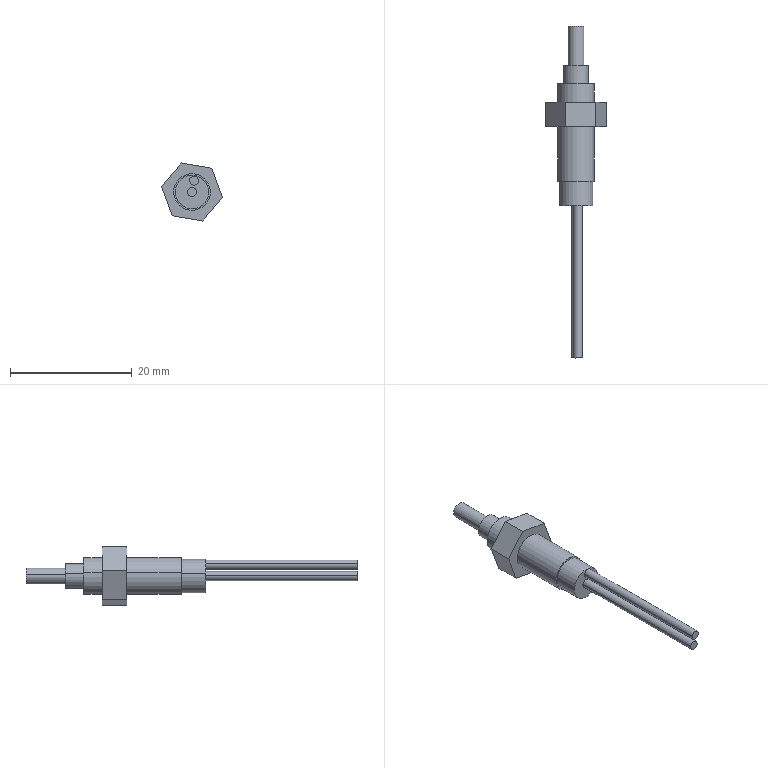Component | SolidWorks | 610FiberOptic-1 | 1 solid | 29 faces | box 10.01 x 54.5 x 9.54 mm | volume 863 mm3 | plane 15 | cylinder 14 | commonest cylinder face diameters 1.5 x4 6 x4 5.5 x2 4 x2 2.6 x2
build123d program:
from build123d import *

# Parameters (mm, degrees)
SKETCH1_R           = 3
BOSS_EXTRUDE1_DEPTH = 20
SKETCH2_R           = 2
BOSS_EXTRUDE2_DEPTH = 3
SKETCH3_R           = 0.75
BOSS_EXTRUDE3_DEPTH = 25
BOSS_EXTRUDE4_DEPTH = 4
SKETCH5_R           = 1.3
BOSS_EXTRUDE5_DEPTH = 11
CUT_EXTRUDE1_START  = -4
SKETCH6_R           = 3
SKETCH6_R_2         = 2.75
CUT_EXTRUDE1_DEPTH  = 4
CUT_EXTRUDE2_START  = -4.5
SKETCH7_R           = 1.3
CUT_EXTRUDE2_DEPTH  = 4.5


with BuildPart() as part:
    # Sketch1 → Boss-Extrude1 (new body)
    with BuildSketch(Plane.XY):
        Circle(SKETCH1_R)
    extrude(amount=BOSS_EXTRUDE1_DEPTH)

    # Sketch2 → Boss-Extrude2 (add)
    with BuildSketch(Plane(origin=(0, 0, 0), x_dir=(-1, 0, 0), z_dir=(0, 0, -1))):
        with Locations(Location((0, 0, 0), (0, 0, 180))):
            Circle(SKETCH2_R)
    extrude(amount=BOSS_EXTRUDE2_DEPTH)

    # Sketch3 → Boss-Extrude3 (add)
    with BuildSketch(Plane.XY.offset(20)):
        with Locations((0, 1.9)):
            Circle(SKETCH3_R)
        Circle(SKETCH3_R)
    extrude(amount=BOSS_EXTRUDE3_DEPTH)

    # Sketch4 → Boss-Extrude4 (add)
    with BuildSketch(Plane(origin=(0, 0, 3), x_dir=(-1, 0, 0), z_dir=(0, 0, -1))):
        Polygon((2.54, 4.4), (-2.54, 4.4), (-5.081, 0), (-2.54, -4.4), (2.54, -4.4), (5.081, 0), align=None)
    extrude(amount=-BOSS_EXTRUDE4_DEPTH)

    # Sketch5 → Boss-Extrude5 (add)
    with BuildSketch(Plane(origin=(0, 0, -3), x_dir=(-1, 0, 0), z_dir=(0, 0, -1))):
        Circle(SKETCH5_R)
    extrude(amount=BOSS_EXTRUDE5_DEPTH)

    # Sketch6 → Cut-Extrude1 (cut)
    with BuildSketch(Plane.XY.offset(20).offset(CUT_EXTRUDE1_START)):
        with Locations(Location((0, 0, 0), (0, 0, 180))):
            Circle(SKETCH6_R)
        Circle(SKETCH6_R_2, mode=Mode.SUBTRACT)
    extrude(amount=CUT_EXTRUDE1_DEPTH, mode=Mode.SUBTRACT)

    # Sketch7 → Cut-Extrude2 (cut)
    with BuildSketch(Plane(origin=(0, 0, -14), x_dir=(-1, 0, 0), z_dir=(0, 0, -1)).offset(CUT_EXTRUDE2_START)):
        Circle(SKETCH7_R)
    extrude(amount=CUT_EXTRUDE2_DEPTH, mode=Mode.SUBTRACT)


solid = part.part

# Placed as in the assembly
solid = solid.moved(Location((-18.365, -4.305, 118.579), (90, 0, -9.806)))
STEP:
#1=CARTESIAN_POINT('',(-0.6939,-1.941,4.663));
#2=VERTEX_POINT('',#1);
#3=CARTESIAN_POINT('',(-0.7521,-1.941,4.673));
#4=VERTEX_POINT('',#3);
#5=CARTESIAN_POINT('',(-0.723,-1.941,4.668));
#6=DIRECTION('',(-0.,-1.,-0.));
#7=DIRECTION('',(0.9854,0.,-0.1703));
#8=AXIS2_PLACEMENT_3D('',#5,#6,#7);
#9=CIRCLE('',#8,0.02953);
#10=EDGE_CURVE('',#2,#4,#9,.T.);
#11=ORIENTED_EDGE('',*,*,#10,.F.);
#12=CARTESIAN_POINT('',(-0.6939,-0.9569,4.663));
#13=VERTEX_POINT('',#12);
#14=CARTESIAN_POINT('',(-0.6939,-1.941,4.663));
#15=DIRECTION('',(0.,1.,0.));
#16=VECTOR('',#15,39.37);
#17=LINE('',#14,#16);
#18=EDGE_CURVE('',#2,#13,#17,.T.);
#19=ORIENTED_EDGE('',*,*,#18,.T.);
#20=CARTESIAN_POINT('',(-0.7521,-0.9569,4.673));
#21=VERTEX_POINT('',#20);
#22=CARTESIAN_POINT('',(-0.723,-0.9569,4.668));
#23=DIRECTION('',(-0.,-1.,-0.));
#24=DIRECTION('',(0.9854,0.,-0.1703));
#25=AXIS2_PLACEMENT_3D('',#22,#23,#24);
#26=CIRCLE('',#25,0.02953);
#27=EDGE_CURVE('',#13,#21,#26,.T.);
#28=ORIENTED_EDGE('',*,*,#27,.T.);
#29=CARTESIAN_POINT('',(-0.7521,-1.941,4.673));
#30=DIRECTION('',(0.,1.,0.));
#31=VECTOR('',#30,39.37);
#32=LINE('',#29,#31);
#33=EDGE_CURVE('',#4,#21,#32,.T.);
#34=ORIENTED_EDGE('',*,*,#33,.F.);
#35=EDGE_LOOP('',(#11,#19,#28,#34));
#36=FACE_OUTER_BOUND('',#35,.T.);
#37=CARTESIAN_POINT('',(-0.723,-1.941,4.668));
#38=DIRECTION('',(0.,1.,0.));
#39=DIRECTION('',(-0.9854,0.,0.1703));
#40=AXIS2_PLACEMENT_3D('',#37,#38,#39);
#41=CYLINDRICAL_SURFACE('',#40,0.02953);
#42=ADVANCED_FACE('',(#36),#41,.T.);
#43=CARTESIAN_POINT('',(-0.6812,-1.941,4.737));
#44=VERTEX_POINT('',#43);
#45=CARTESIAN_POINT('',(-0.7394,-1.941,4.747));
#46=VERTEX_POINT('',#45);
#47=CARTESIAN_POINT('',(-0.7103,-1.941,4.742));
#48=DIRECTION('',(-0.,-1.,-0.));
#49=DIRECTION('',(0.9854,0.,-0.1703));
#50=AXIS2_PLACEMENT_3D('',#47,#48,#49);
#51=CIRCLE('',#50,0.02953);
#52=EDGE_CURVE('',#44,#46,#51,.T.);
#53=ORIENTED_EDGE('',*,*,#52,.F.);
#54=CARTESIAN_POINT('',(-0.6812,-0.9569,4.737));
#55=VERTEX_POINT('',#54);
#56=CARTESIAN_POINT('',(-0.6812,-1.941,4.737));
#57=DIRECTION('',(0.,1.,0.));
#58=VECTOR('',#57,39.37);
#59=LINE('',#56,#58);
#60=EDGE_CURVE('',#44,#55,#59,.T.);
#61=ORIENTED_EDGE('',*,*,#60,.T.);
#62=CARTESIAN_POINT('',(-0.7394,-0.9569,4.747));
#63=VERTEX_POINT('',#62);
#64=CARTESIAN_POINT('',(-0.7103,-0.9569,4.742));
#65=DIRECTION('',(-0.,-1.,-0.));
#66=DIRECTION('',(0.9854,0.,-0.1703));
#67=AXIS2_PLACEMENT_3D('',#64,#65,#66);
#68=CIRCLE('',#67,0.02953);
#69=EDGE_CURVE('',#55,#63,#68,.T.);
#70=ORIENTED_EDGE('',*,*,#69,.T.);
#71=CARTESIAN_POINT('',(-0.7394,-1.941,4.747));
#72=DIRECTION('',(0.,1.,0.));
#73=VECTOR('',#72,39.37);
#74=LINE('',#71,#73);
#75=EDGE_CURVE('',#46,#63,#74,.T.);
#76=ORIENTED_EDGE('',*,*,#75,.F.);
#77=EDGE_LOOP('',(#53,#61,#70,#76));
#78=FACE_OUTER_BOUND('',#77,.T.);
#79=CARTESIAN_POINT('',(-0.7103,-1.941,4.742));
#80=DIRECTION('',(0.,1.,0.));
#81=DIRECTION('',(-0.9854,0.,0.1703));
#82=AXIS2_PLACEMENT_3D('',#79,#80,#81);
#83=CYLINDRICAL_SURFACE('',#82,0.02953);
#84=ADVANCED_FACE('',(#78),#83,.T.);
#85=CARTESIAN_POINT('',(-0.6163,-0.7994,4.65));
#86=VERTEX_POINT('',#85);
#87=CARTESIAN_POINT('',(-0.8297,-0.7994,4.687));
#88=VERTEX_POINT('',#87);
#89=CARTESIAN_POINT('',(-0.723,-0.7994,4.668));
#90=DIRECTION('',(-0.,-1.,-0.));
#91=DIRECTION('',(0.9854,0.,-0.1703));
#92=AXIS2_PLACEMENT_3D('',#89,#90,#91);
#93=CIRCLE('',#92,0.1083);
#94=EDGE_CURVE('',#86,#88,#93,.T.);
#95=ORIENTED_EDGE('',*,*,#94,.T.);
#96=CARTESIAN_POINT('',(-0.8297,-0.9569,4.687));
#97=VERTEX_POINT('',#96);
#98=CARTESIAN_POINT('',(-0.8297,-0.7994,4.687));
#99=DIRECTION('',(-0.,-1.,-0.));
#100=VECTOR('',#99,39.37);
#101=LINE('',#98,#100);
#102=EDGE_CURVE('',#88,#97,#101,.T.);
#103=ORIENTED_EDGE('',*,*,#102,.T.);
#104=CARTESIAN_POINT('',(-0.6163,-0.9569,4.65));
#105=VERTEX_POINT('',#104);
#106=CARTESIAN_POINT('',(-0.723,-0.9569,4.668));
#107=DIRECTION('',(-0.,-1.,-0.));
#108=DIRECTION('',(0.9854,0.,-0.1703));
#109=AXIS2_PLACEMENT_3D('',#106,#107,#108);
#110=CIRCLE('',#109,0.1083);
#111=EDGE_CURVE('',#105,#97,#110,.T.);
#112=ORIENTED_EDGE('',*,*,#111,.F.);
#113=CARTESIAN_POINT('',(-0.6163,-0.7994,4.65));
#114=DIRECTION('',(-0.,-1.,-0.));
#115=VECTOR('',#114,39.37);
#116=LINE('',#113,#115);
#117=EDGE_CURVE('',#86,#105,#116,.T.);
#118=ORIENTED_EDGE('',*,*,#117,.F.);
#119=EDGE_LOOP('',(#95,#103,#112,#118));
#120=FACE_OUTER_BOUND('',#119,.T.);
#121=CARTESIAN_POINT('',(-0.723,-0.7994,4.668));
#122=DIRECTION('',(-0.,-1.,-0.));
#123=DIRECTION('',(0.9854,0.,-0.1703));
#124=AXIS2_PLACEMENT_3D('',#121,#122,#123);
#125=CYLINDRICAL_SURFACE('',#124,0.1083);
#126=ADVANCED_FACE('',(#120),#125,.T.);
#127=CARTESIAN_POINT('',(-0.8394,-0.2876,4.689));
#128=VERTEX_POINT('',#127);
#129=CARTESIAN_POINT('',(-0.6067,-0.2876,4.648));
#130=VERTEX_POINT('',#129);
#131=CARTESIAN_POINT('',(-0.723,-0.2876,4.668));
#132=DIRECTION('',(0.,1.,0.));
#133=DIRECTION('',(-0.9854,0.,0.1703));
#134=AXIS2_PLACEMENT_3D('',#131,#132,#133);
#135=CIRCLE('',#134,0.1181);
#136=EDGE_CURVE('',#128,#130,#135,.T.);
#137=ORIENTED_EDGE('',*,*,#136,.T.);
#138=CARTESIAN_POINT('',(-0.6067,-0.1695,4.648));
#139=VERTEX_POINT('',#138);
#140=CARTESIAN_POINT('',(-0.6067,-0.9569,4.648));
#141=DIRECTION('',(0.,1.,0.));
#142=VECTOR('',#141,39.37);
#143=LINE('',#140,#142);
#144=EDGE_CURVE('',#130,#139,#143,.T.);
#145=ORIENTED_EDGE('',*,*,#144,.T.);
#146=CARTESIAN_POINT('',(-0.8394,-0.1695,4.689));
#147=VERTEX_POINT('',#146);
#148=CARTESIAN_POINT('',(-0.723,-0.1695,4.668));
#149=DIRECTION('',(-0.,-1.,-0.));
#150=DIRECTION('',(0.9854,0.,-0.1703));
#151=AXIS2_PLACEMENT_3D('',#148,#149,#150);
#152=CIRCLE('',#151,0.1181);
#153=EDGE_CURVE('',#139,#147,#152,.T.);
#154=ORIENTED_EDGE('',*,*,#153,.T.);
#155=CARTESIAN_POINT('',(-0.8394,-0.9569,4.689));
#156=DIRECTION('',(0.,1.,0.));
#157=VECTOR('',#156,39.37);
#158=LINE('',#155,#157);
#159=EDGE_CURVE('',#128,#147,#158,.T.);
#160=ORIENTED_EDGE('',*,*,#159,.F.);
#161=EDGE_LOOP('',(#137,#145,#154,#160));
#162=FACE_OUTER_BOUND('',#161,.T.);
#163=CARTESIAN_POINT('',(-0.723,-0.9569,4.668));
#164=DIRECTION('',(0.,1.,0.));
#165=DIRECTION('',(-0.9854,0.,0.1703));
#166=AXIS2_PLACEMENT_3D('',#163,#164,#165);
#167=CYLINDRICAL_SURFACE('',#166,0.1181);
#168=ADVANCED_FACE('',(#162),#167,.T.);
#169=CARTESIAN_POINT('',(-0.8006,-0.05139,4.682));
#170=VERTEX_POINT('',#169);
#171=CARTESIAN_POINT('',(-0.6454,-0.05139,4.655));
#172=VERTEX_POINT('',#171);
#173=CARTESIAN_POINT('',(-0.723,-0.05139,4.668));
#174=DIRECTION('',(0.,1.,0.));
#175=DIRECTION('',(-0.9854,0.,0.1703));
#176=AXIS2_PLACEMENT_3D('',#173,#174,#175);
#177=CIRCLE('',#176,0.07874);
#178=EDGE_CURVE('',#170,#172,#177,.T.);
#179=ORIENTED_EDGE('',*,*,#178,.F.);
#180=CARTESIAN_POINT('',(-0.8006,-0.1695,4.682));
#181=VERTEX_POINT('',#180);
#182=CARTESIAN_POINT('',(-0.8006,-0.05139,4.682));
#183=DIRECTION('',(-0.,-1.,-0.));
#184=VECTOR('',#183,39.37);
#185=LINE('',#182,#184);
#186=EDGE_CURVE('',#170,#181,#185,.T.);
#187=ORIENTED_EDGE('',*,*,#186,.T.);
#188=CARTESIAN_POINT('',(-0.6454,-0.1695,4.655));
#189=VERTEX_POINT('',#188);
#190=CARTESIAN_POINT('',(-0.723,-0.1695,4.668));
#191=DIRECTION('',(0.,1.,0.));
#192=DIRECTION('',(0.9854,0.,-0.1703));
#193=AXIS2_PLACEMENT_3D('',#190,#191,#192);
#194=CIRCLE('',#193,0.07874);
#195=EDGE_CURVE('',#181,#189,#194,.T.);
#196=ORIENTED_EDGE('',*,*,#195,.T.);
#197=CARTESIAN_POINT('',(-0.6454,-0.05139,4.655));
#198=DIRECTION('',(-0.,-1.,-0.));
#199=VECTOR('',#198,39.37);
#200=LINE('',#197,#199);
#201=EDGE_CURVE('',#172,#189,#200,.T.);
#202=ORIENTED_EDGE('',*,*,#201,.F.);
#203=EDGE_LOOP('',(#179,#187,#196,#202));
#204=FACE_OUTER_BOUND('',#203,.T.);
#205=CARTESIAN_POINT('',(-0.723,-0.05139,4.668));
#206=DIRECTION('',(-0.,-1.,-0.));
#207=DIRECTION('',(0.9854,0.,-0.1703));
#208=AXIS2_PLACEMENT_3D('',#205,#206,#207);
#209=CYLINDRICAL_SURFACE('',#208,0.07874);
#210=ADVANCED_FACE('',(#204),#209,.T.);
#211=CARTESIAN_POINT('',(-0.6067,-0.7994,4.648));
#212=VERTEX_POINT('',#211);
#213=CARTESIAN_POINT('',(-0.8394,-0.7994,4.689));
#214=VERTEX_POINT('',#213);
#215=CARTESIAN_POINT('',(-0.723,-0.7994,4.668));
#216=DIRECTION('',(-0.,-1.,-0.));
#217=DIRECTION('',(0.9854,0.,-0.1703));
#218=AXIS2_PLACEMENT_3D('',#215,#216,#217);
#219=CIRCLE('',#218,0.1181);
#220=EDGE_CURVE('',#212,#214,#219,.T.);
#221=ORIENTED_EDGE('',*,*,#220,.F.);
#222=CARTESIAN_POINT('',(-0.6067,-0.4451,4.648));
#223=VERTEX_POINT('',#222);
#224=CARTESIAN_POINT('',(-0.6067,-0.9569,4.648));
#225=DIRECTION('',(0.,1.,0.));
#226=VECTOR('',#225,39.37);
#227=LINE('',#224,#226);
#228=EDGE_CURVE('',#212,#223,#227,.T.);
#229=ORIENTED_EDGE('',*,*,#228,.T.);
#230=CARTESIAN_POINT('',(-0.8394,-0.4451,4.689));
#231=VERTEX_POINT('',#230);
#232=CARTESIAN_POINT('',(-0.723,-0.4451,4.668));
#233=DIRECTION('',(0.,1.,0.));
#234=DIRECTION('',(-0.9854,0.,0.1703));
#235=AXIS2_PLACEMENT_3D('',#232,#233,#234);
#236=CIRCLE('',#235,0.1181);
#237=EDGE_CURVE('',#231,#223,#236,.T.);
#238=ORIENTED_EDGE('',*,*,#237,.F.);
#239=CARTESIAN_POINT('',(-0.8394,-0.9569,4.689));
#240=DIRECTION('',(0.,1.,0.));
#241=VECTOR('',#240,39.37);
#242=LINE('',#239,#241);
#243=EDGE_CURVE('',#214,#231,#242,.T.);
#244=ORIENTED_EDGE('',*,*,#243,.F.);
#245=EDGE_LOOP('',(#221,#229,#238,#244));
#246=FACE_OUTER_BOUND('',#245,.T.);
#247=CARTESIAN_POINT('',(-0.723,-0.9569,4.668));
#248=DIRECTION('',(0.,1.,0.));
#249=DIRECTION('',(-0.9854,0.,0.1703));
#250=AXIS2_PLACEMENT_3D('',#247,#248,#249);
#251=CYLINDRICAL_SURFACE('',#250,0.1181);
#252=ADVANCED_FACE('',(#246),#251,.T.);
#253=CARTESIAN_POINT('',(-0.7735,0.2045,4.677));
#254=VERTEX_POINT('',#253);
#255=CARTESIAN_POINT('',(-0.6726,0.2045,4.66));
#256=VERTEX_POINT('',#255);
#257=CARTESIAN_POINT('',(-0.723,0.2045,4.668));
#258=DIRECTION('',(0.,1.,0.));
#259=DIRECTION('',(-0.9854,0.,0.1703));
#260=AXIS2_PLACEMENT_3D('',#257,#258,#259);
#261=CIRCLE('',#260,0.05118);
#262=EDGE_CURVE('',#254,#256,#261,.T.);
#263=ORIENTED_EDGE('',*,*,#262,.F.);
#264=CARTESIAN_POINT('',(-0.7735,-0.05139,4.677));
#265=VERTEX_POINT('',#264);
#266=CARTESIAN_POINT('',(-0.7735,0.3817,4.677));
#267=DIRECTION('',(-0.,-1.,-0.));
#268=VECTOR('',#267,39.37);
#269=LINE('',#266,#268);
#270=EDGE_CURVE('',#254,#265,#269,.T.);
#271=ORIENTED_EDGE('',*,*,#270,.T.);
#272=CARTESIAN_POINT('',(-0.6726,-0.05139,4.66));
#273=VERTEX_POINT('',#272);
#274=CARTESIAN_POINT('',(-0.723,-0.05139,4.668));
#275=DIRECTION('',(0.,1.,0.));
#276=DIRECTION('',(-0.9854,0.,0.1703));
#277=AXIS2_PLACEMENT_3D('',#274,#275,#276);
#278=CIRCLE('',#277,0.05118);
#279=EDGE_CURVE('',#265,#273,#278,.T.);
#280=ORIENTED_EDGE('',*,*,#279,.T.);
#281=CARTESIAN_POINT('',(-0.6726,0.3817,4.66));
#282=DIRECTION('',(-0.,-1.,-0.));
#283=VECTOR('',#282,39.37);
#284=LINE('',#281,#283);
#285=EDGE_CURVE('',#256,#273,#284,.T.);
#286=ORIENTED_EDGE('',*,*,#285,.F.);
#287=EDGE_LOOP('',(#263,#271,#280,#286));
#288=FACE_OUTER_BOUND('',#287,.T.);
#289=CARTESIAN_POINT('',(-0.723,0.3817,4.668));
#290=DIRECTION('',(-0.,-1.,-0.));
#291=DIRECTION('',(0.9854,0.,-0.1703));
#292=AXIS2_PLACEMENT_3D('',#289,#290,#291);
#293=CYLINDRICAL_SURFACE('',#292,0.05118);
#294=ADVANCED_FACE('',(#288),#293,.T.);
#295=ORIENTED_EDGE('',*,*,#270,.F.);
#296=CARTESIAN_POINT('',(-0.723,0.2045,4.668));
#297=DIRECTION('',(0.,1.,0.));
#298=DIRECTION('',(-0.9854,0.,0.1703));
#299=AXIS2_PLACEMENT_3D('',#296,#297,#298);
#300=CIRCLE('',#299,0.05118);
#301=EDGE_CURVE('',#256,#254,#300,.T.);
#302=ORIENTED_EDGE('',*,*,#301,.F.);
#303=ORIENTED_EDGE('',*,*,#285,.T.);
#304=CARTESIAN_POINT('',(-0.723,-0.05139,4.668));
#305=DIRECTION('',(0.,1.,0.));
#306=DIRECTION('',(-0.9854,0.,0.1703));
#307=AXIS2_PLACEMENT_3D('',#304,#305,#306);
#308=CIRCLE('',#307,0.05118);
#309=EDGE_CURVE('',#273,#265,#308,.T.);
#310=ORIENTED_EDGE('',*,*,#309,.T.);
#311=EDGE_LOOP('',(#295,#302,#303,#310));
#312=FACE_OUTER_BOUND('',#311,.T.);
#313=CARTESIAN_POINT('',(-0.723,0.3817,4.668));
#314=DIRECTION('',(-0.,-1.,-0.));
#315=DIRECTION('',(0.9854,0.,-0.1703));
#316=AXIS2_PLACEMENT_3D('',#313,#314,#315);
#317=CYLINDRICAL_SURFACE('',#316,0.05118);
#318=ADVANCED_FACE('',(#312),#317,.T.);
#319=ORIENTED_EDGE('',*,*,#228,.F.);
#320=CARTESIAN_POINT('',(-0.723,-0.7994,4.668));
#321=DIRECTION('',(-0.,-1.,-0.));
#322=DIRECTION('',(0.9854,0.,-0.1703));
#323=AXIS2_PLACEMENT_3D('',#320,#321,#322);
#324=CIRCLE('',#323,0.1181);
#325=EDGE_CURVE('',#214,#212,#324,.T.);
#326=ORIENTED_EDGE('',*,*,#325,.F.);
#327=ORIENTED_EDGE('',*,*,#243,.T.);
#328=CARTESIAN_POINT('',(-0.723,-0.4451,4.668));
#329=DIRECTION('',(0.,1.,0.));
#330=DIRECTION('',(-0.9854,0.,0.1703));
#331=AXIS2_PLACEMENT_3D('',#328,#329,#330);
#332=CIRCLE('',#331,0.1181);
#333=EDGE_CURVE('',#223,#231,#332,.T.);
#334=ORIENTED_EDGE('',*,*,#333,.F.);
#335=EDGE_LOOP('',(#319,#326,#327,#334));
#336=FACE_OUTER_BOUND('',#335,.T.);
#337=CARTESIAN_POINT('',(-0.723,-0.9569,4.668));
#338=DIRECTION('',(0.,1.,0.));
#339=DIRECTION('',(-0.9854,0.,0.1703));
#340=AXIS2_PLACEMENT_3D('',#337,#338,#339);
#341=CYLINDRICAL_SURFACE('',#340,0.1181);
#342=ADVANCED_FACE('',(#336),#341,.T.);
#343=CARTESIAN_POINT('',(-0.723,-0.05139,4.668));
#344=DIRECTION('',(0.,1.,0.));
#345=DIRECTION('',(-0.9854,0.,0.1703));
#346=AXIS2_PLACEMENT_3D('',#343,#344,#345);
#347=CIRCLE('',#346,0.07874);
#348=EDGE_CURVE('',#172,#170,#347,.T.);
#349=ORIENTED_EDGE('',*,*,#348,.T.);
#350=ORIENTED_EDGE('',*,*,#178,.T.);
#351=EDGE_LOOP('',(#349,#350));
#352=FACE_OUTER_BOUND('',#351,.T.);
#353=ORIENTED_EDGE('',*,*,#309,.F.);
#354=ORIENTED_EDGE('',*,*,#279,.F.);
#355=EDGE_LOOP('',(#353,#354));
#356=FACE_BOUND('',#355,.T.);
#357=CARTESIAN_POINT('',(-0.723,-0.05139,4.668));
#358=DIRECTION('',(0.,1.,0.));
#359=DIRECTION('',(-0.9854,0.,0.1703));
#360=AXIS2_PLACEMENT_3D('',#357,#358,#359);
#361=PLANE('',#360);
#362=ADVANCED_FACE('',(#352,#356),#361,.T.);
#363=CARTESIAN_POINT('',(-0.9201,-0.4451,4.703));
#364=VERTEX_POINT('',#363);
#365=CARTESIAN_POINT('',(-0.7921,-0.4451,4.856));
#366=VERTEX_POINT('',#365);
#367=CARTESIAN_POINT('',(-0.9201,-0.4451,4.703));
#368=DIRECTION('',(0.6402,-0.,0.7682));
#369=VECTOR('',#368,39.37);
#370=LINE('',#367,#369);
#371=EDGE_CURVE('',#364,#366,#370,.T.);
#372=ORIENTED_EDGE('',*,*,#371,.F.);
#373=CARTESIAN_POINT('',(-0.8511,-0.4451,4.515));
#374=VERTEX_POINT('',#373);
#375=CARTESIAN_POINT('',(-0.8511,-0.4451,4.515));
#376=DIRECTION('',(-0.3452,-0.,0.9385));
#377=VECTOR('',#376,39.37);
#378=LINE('',#375,#377);
#379=EDGE_CURVE('',#374,#364,#378,.T.);
#380=ORIENTED_EDGE('',*,*,#379,.F.);
#381=CARTESIAN_POINT('',(-0.654,-0.4451,4.481));
#382=VERTEX_POINT('',#381);
#383=CARTESIAN_POINT('',(-0.654,-0.4451,4.481));
#384=DIRECTION('',(-0.9854,0.,0.1703));
#385=VECTOR('',#384,39.37);
#386=LINE('',#383,#385);
#387=EDGE_CURVE('',#382,#374,#386,.T.);
#388=ORIENTED_EDGE('',*,*,#387,.F.);
#389=CARTESIAN_POINT('',(-0.5259,-0.4451,4.634));
#390=VERTEX_POINT('',#389);
#391=CARTESIAN_POINT('',(-0.5259,-0.4451,4.634));
#392=DIRECTION('',(-0.6402,0.,-0.7682));
#393=VECTOR('',#392,39.37);
#394=LINE('',#391,#393);
#395=EDGE_CURVE('',#390,#382,#394,.T.);
#396=ORIENTED_EDGE('',*,*,#395,.F.);
#397=CARTESIAN_POINT('',(-0.595,-0.4451,4.822));
#398=VERTEX_POINT('',#397);
#399=CARTESIAN_POINT('',(-0.595,-0.4451,4.822));
#400=DIRECTION('',(0.3452,0.,-0.9385));
#401=VECTOR('',#400,39.37);
#402=LINE('',#399,#401);
#403=EDGE_CURVE('',#398,#390,#402,.T.);
#404=ORIENTED_EDGE('',*,*,#403,.F.);
#405=CARTESIAN_POINT('',(-0.7921,-0.4451,4.856));
#406=DIRECTION('',(0.9854,-0.,-0.1703));
#407=VECTOR('',#406,39.37);
#408=LINE('',#405,#407);
#409=EDGE_CURVE('',#366,#398,#408,.T.);
#410=ORIENTED_EDGE('',*,*,#409,.F.);
#411=EDGE_LOOP('',(#372,#380,#388,#396,#404,#410));
#412=FACE_OUTER_BOUND('',#411,.T.);
#413=ORIENTED_EDGE('',*,*,#237,.T.);
#414=ORIENTED_EDGE('',*,*,#333,.T.);
#415=EDGE_LOOP('',(#413,#414));
#416=FACE_BOUND('',#415,.T.);
#417=CARTESIAN_POINT('',(-0.723,-0.4451,4.668));
#418=DIRECTION('',(0.,1.,0.));
#419=DIRECTION('',(-0.9854,0.,0.1703));
#420=AXIS2_PLACEMENT_3D('',#417,#418,#419);
#421=PLANE('',#420);
#422=ADVANCED_FACE('',(#412,#416),#421,.F.);
#423=CARTESIAN_POINT('',(-0.9201,-0.2876,4.703));
#424=VERTEX_POINT('',#423);
#425=CARTESIAN_POINT('',(-0.7921,-0.2876,4.856));
#426=VERTEX_POINT('',#425);
#427=CARTESIAN_POINT('',(-0.9201,-0.2876,4.703));
#428=DIRECTION('',(0.6402,-0.,0.7682));
#429=VECTOR('',#428,39.37);
#430=LINE('',#427,#429);
#431=EDGE_CURVE('',#424,#426,#430,.T.);
#432=ORIENTED_EDGE('',*,*,#431,.T.);
#433=CARTESIAN_POINT('',(-0.595,-0.2876,4.822));
#434=VERTEX_POINT('',#433);
#435=CARTESIAN_POINT('',(-0.7921,-0.2876,4.856));
#436=DIRECTION('',(0.9854,-0.,-0.1703));
#437=VECTOR('',#436,39.37);
#438=LINE('',#435,#437);
#439=EDGE_CURVE('',#426,#434,#438,.T.);
#440=ORIENTED_EDGE('',*,*,#439,.T.);
#441=CARTESIAN_POINT('',(-0.5259,-0.2876,4.634));
#442=VERTEX_POINT('',#441);
#443=CARTESIAN_POINT('',(-0.595,-0.2876,4.822));
#444=DIRECTION('',(0.3452,0.,-0.9385));
#445=VECTOR('',#444,39.37);
#446=LINE('',#443,#445);
#447=EDGE_CURVE('',#434,#442,#446,.T.);
#448=ORIENTED_EDGE('',*,*,#447,.T.);
#449=CARTESIAN_POINT('',(-0.654,-0.2876,4.481));
#450=VERTEX_POINT('',#449);
#451=CARTESIAN_POINT('',(-0.5259,-0.2876,4.634));
#452=DIRECTION('',(-0.6402,0.,-0.7682));
#453=VECTOR('',#452,39.37);
#454=LINE('',#451,#453);
#455=EDGE_CURVE('',#442,#450,#454,.T.);
#456=ORIENTED_EDGE('',*,*,#455,.T.);
#457=CARTESIAN_POINT('',(-0.8511,-0.2876,4.515));
#458=VERTEX_POINT('',#457);
#459=CARTESIAN_POINT('',(-0.654,-0.2876,4.481));
#460=DIRECTION('',(-0.9854,0.,0.1703));
#461=VECTOR('',#460,39.37);
#462=LINE('',#459,#461);
#463=EDGE_CURVE('',#450,#458,#462,.T.);
#464=ORIENTED_EDGE('',*,*,#463,.T.);
#465=CARTESIAN_POINT('',(-0.8511,-0.2876,4.515));
#466=DIRECTION('',(-0.3452,-0.,0.9385));
#467=VECTOR('',#466,39.37);
#468=LINE('',#465,#467);
#469=EDGE_CURVE('',#458,#424,#468,.T.);
#470=ORIENTED_EDGE('',*,*,#469,.T.);
#471=EDGE_LOOP('',(#432,#440,#448,#456,#464,#470));
#472=FACE_OUTER_BOUND('',#471,.T.);
#473=ORIENTED_EDGE('',*,*,#136,.F.);
#474=CARTESIAN_POINT('',(-0.723,-0.2876,4.668));
#475=DIRECTION('',(0.,1.,0.));
#476=DIRECTION('',(-0.9854,0.,0.1703));
#477=AXIS2_PLACEMENT_3D('',#474,#475,#476);
#478=CIRCLE('',#477,0.1181);
#479=EDGE_CURVE('',#130,#128,#478,.T.);
#480=ORIENTED_EDGE('',*,*,#479,.F.);
#481=EDGE_LOOP('',(#473,#480));
#482=FACE_BOUND('',#481,.T.);
#483=CARTESIAN_POINT('',(-0.723,-0.2876,4.668));
#484=DIRECTION('',(0.,1.,0.));
#485=DIRECTION('',(-0.9854,0.,0.1703));
#486=AXIS2_PLACEMENT_3D('',#483,#484,#485);
#487=PLANE('',#486);
#488=ADVANCED_FACE('',(#472,#482),#487,.T.);
#489=ORIENTED_EDGE('',*,*,#431,.F.);
#490=CARTESIAN_POINT('',(-0.9201,-0.4451,4.703));
#491=DIRECTION('',(0.,1.,0.));
#492=VECTOR('',#491,39.37);
#493=LINE('',#490,#492);
#494=EDGE_CURVE('',#364,#424,#493,.T.);
#495=ORIENTED_EDGE('',*,*,#494,.F.);
#496=ORIENTED_EDGE('',*,*,#371,.T.);
#497=CARTESIAN_POINT('',(-0.7921,-0.4451,4.856));
#498=DIRECTION('',(0.,1.,0.));
#499=VECTOR('',#498,39.37);
#500=LINE('',#497,#499);
#501=EDGE_CURVE('',#366,#426,#500,.T.);
#502=ORIENTED_EDGE('',*,*,#501,.T.);
#503=EDGE_LOOP('',(#489,#495,#496,#502));
#504=FACE_OUTER_BOUND('',#503,.T.);
#505=CARTESIAN_POINT('',(-0.9201,-0.4451,4.703));
#506=DIRECTION('',(-0.7682,0.,0.6402));
#507=DIRECTION('',(-0.6402,0.,-0.7682));
#508=AXIS2_PLACEMENT_3D('',#505,#506,#507);
#509=PLANE('',#508);
#510=ADVANCED_FACE('',(#504),#509,.T.);
#511=ORIENTED_EDGE('',*,*,#469,.F.);
#512=CARTESIAN_POINT('',(-0.8511,-0.4451,4.515));
#513=DIRECTION('',(0.,1.,0.));
#514=VECTOR('',#513,39.37);
#515=LINE('',#512,#514);
#516=EDGE_CURVE('',#374,#458,#515,.T.);
#517=ORIENTED_EDGE('',*,*,#516,.F.);
#518=ORIENTED_EDGE('',*,*,#379,.T.);
#519=ORIENTED_EDGE('',*,*,#494,.T.);
#520=EDGE_LOOP('',(#511,#517,#518,#519));
#521=FACE_OUTER_BOUND('',#520,.T.);
#522=CARTESIAN_POINT('',(-0.8511,-0.4451,4.515));
#523=DIRECTION('',(-0.9385,0.,-0.3452));
#524=DIRECTION('',(0.3452,0.,-0.9385));
#525=AXIS2_PLACEMENT_3D('',#522,#523,#524);
#526=PLANE('',#525);
#527=ADVANCED_FACE('',(#521),#526,.T.);
#528=ORIENTED_EDGE('',*,*,#463,.F.);
#529=CARTESIAN_POINT('',(-0.654,-0.4451,4.481));
#530=DIRECTION('',(0.,1.,0.));
#531=VECTOR('',#530,39.37);
#532=LINE('',#529,#531);
#533=EDGE_CURVE('',#382,#450,#532,.T.);
#534=ORIENTED_EDGE('',*,*,#533,.F.);
#535=ORIENTED_EDGE('',*,*,#387,.T.);
#536=ORIENTED_EDGE('',*,*,#516,.T.);
#537=EDGE_LOOP('',(#528,#534,#535,#536));
#538=FACE_OUTER_BOUND('',#537,.T.);
#539=CARTESIAN_POINT('',(-0.654,-0.4451,4.481));
#540=DIRECTION('',(-0.1703,0.,-0.9854));
#541=DIRECTION('',(0.9854,-0.,-0.1703));
#542=AXIS2_PLACEMENT_3D('',#539,#540,#541);
#543=PLANE('',#542);
#544=ADVANCED_FACE('',(#538),#543,.T.);
#545=ORIENTED_EDGE('',*,*,#455,.F.);
#546=CARTESIAN_POINT('',(-0.5259,-0.4451,4.634));
#547=DIRECTION('',(0.,1.,0.));
#548=VECTOR('',#547,39.37);
#549=LINE('',#546,#548);
#550=EDGE_CURVE('',#390,#442,#549,.T.);
#551=ORIENTED_EDGE('',*,*,#550,.F.);
#552=ORIENTED_EDGE('',*,*,#395,.T.);
#553=ORIENTED_EDGE('',*,*,#533,.T.);
#554=EDGE_LOOP('',(#545,#551,#552,#553));
#555=FACE_OUTER_BOUND('',#554,.T.);
#556=CARTESIAN_POINT('',(-0.5259,-0.4451,4.634));
#557=DIRECTION('',(0.7682,-0.,-0.6402));
#558=DIRECTION('',(0.6402,-0.,0.7682));
#559=AXIS2_PLACEMENT_3D('',#556,#557,#558);
#560=PLANE('',#559);
#561=ADVANCED_FACE('',(#555),#560,.T.);
#562=ORIENTED_EDGE('',*,*,#447,.F.);
#563=CARTESIAN_POINT('',(-0.595,-0.4451,4.822));
#564=DIRECTION('',(0.,1.,0.));
#565=VECTOR('',#564,39.37);
#566=LINE('',#563,#565);
#567=EDGE_CURVE('',#398,#434,#566,.T.);
#568=ORIENTED_EDGE('',*,*,#567,.F.);
#569=ORIENTED_EDGE('',*,*,#403,.T.);
#570=ORIENTED_EDGE('',*,*,#550,.T.);
#571=EDGE_LOOP('',(#562,#568,#569,#570));
#572=FACE_OUTER_BOUND('',#571,.T.);
#573=CARTESIAN_POINT('',(-0.595,-0.4451,4.822));
#574=DIRECTION('',(0.9385,-0.,0.3452));
#575=DIRECTION('',(-0.3452,-0.,0.9385));
#576=AXIS2_PLACEMENT_3D('',#573,#574,#575);
#577=PLANE('',#576);
#578=ADVANCED_FACE('',(#572),#577,.T.);
#579=ORIENTED_EDGE('',*,*,#439,.F.);
#580=ORIENTED_EDGE('',*,*,#501,.F.);
#581=ORIENTED_EDGE('',*,*,#409,.T.);
#582=ORIENTED_EDGE('',*,*,#567,.T.);
#583=EDGE_LOOP('',(#579,#580,#581,#582));
#584=FACE_OUTER_BOUND('',#583,.T.);
#585=CARTESIAN_POINT('',(-0.7921,-0.4451,4.856));
#586=DIRECTION('',(0.1703,-0.,0.9854));
#587=DIRECTION('',(-0.9854,0.,0.1703));
#588=AXIS2_PLACEMENT_3D('',#585,#586,#587);
#589=PLANE('',#588);
#590=ADVANCED_FACE('',(#584),#589,.T.);
#591=ORIENTED_EDGE('',*,*,#186,.F.);
#592=ORIENTED_EDGE('',*,*,#348,.F.);
#593=ORIENTED_EDGE('',*,*,#201,.T.);
#594=CARTESIAN_POINT('',(-0.723,-0.1695,4.668));
#595=DIRECTION('',(0.,1.,0.));
#596=DIRECTION('',(0.9854,0.,-0.1703));
#597=AXIS2_PLACEMENT_3D('',#594,#595,#596);
#598=CIRCLE('',#597,0.07874);
#599=EDGE_CURVE('',#189,#181,#598,.T.);
#600=ORIENTED_EDGE('',*,*,#599,.T.);
#601=EDGE_LOOP('',(#591,#592,#593,#600));
#602=FACE_OUTER_BOUND('',#601,.T.);
#603=CARTESIAN_POINT('',(-0.723,-0.05139,4.668));
#604=DIRECTION('',(-0.,-1.,-0.));
#605=DIRECTION('',(0.9854,0.,-0.1703));
#606=AXIS2_PLACEMENT_3D('',#603,#604,#605);
#607=CYLINDRICAL_SURFACE('',#606,0.07874);
#608=ADVANCED_FACE('',(#602),#607,.T.);
#609=CARTESIAN_POINT('',(-0.723,-0.1695,4.668));
#610=DIRECTION('',(-0.,-1.,-0.));
#611=DIRECTION('',(0.9854,0.,-0.1703));
#612=AXIS2_PLACEMENT_3D('',#609,#610,#611);
#613=CIRCLE('',#612,0.1181);
#614=EDGE_CURVE('',#147,#139,#613,.T.);
#615=ORIENTED_EDGE('',*,*,#614,.F.);
#616=ORIENTED_EDGE('',*,*,#153,.F.);
#617=EDGE_LOOP('',(#615,#616));
#618=FACE_OUTER_BOUND('',#617,.T.);
#619=ORIENTED_EDGE('',*,*,#599,.F.);
#620=ORIENTED_EDGE('',*,*,#195,.F.);
#621=EDGE_LOOP('',(#619,#620));
#622=FACE_BOUND('',#621,.T.);
#623=CARTESIAN_POINT('',(-0.723,-0.1695,4.668));
#624=DIRECTION('',(-0.,-1.,-0.));
#625=DIRECTION('',(0.9854,-0.,-0.1703));
#626=AXIS2_PLACEMENT_3D('',#623,#624,#625);
#627=PLANE('',#626);
#628=ADVANCED_FACE('',(#618,#622),#627,.F.);
#629=ORIENTED_EDGE('',*,*,#144,.F.);
#630=ORIENTED_EDGE('',*,*,#479,.T.);
#631=ORIENTED_EDGE('',*,*,#159,.T.);
#632=ORIENTED_EDGE('',*,*,#614,.T.);
#633=EDGE_LOOP('',(#629,#630,#631,#632));
#634=FACE_OUTER_BOUND('',#633,.T.);
#635=CARTESIAN_POINT('',(-0.723,-0.9569,4.668));
#636=DIRECTION('',(0.,1.,0.));
#637=DIRECTION('',(-0.9854,0.,0.1703));
#638=AXIS2_PLACEMENT_3D('',#635,#636,#637);
#639=CYLINDRICAL_SURFACE('',#638,0.1181);
#640=ADVANCED_FACE('',(#634),#639,.T.);
#641=ORIENTED_EDGE('',*,*,#94,.F.);
#642=CARTESIAN_POINT('',(-0.723,-0.7994,4.668));
#643=DIRECTION('',(-0.,-1.,-0.));
#644=DIRECTION('',(0.9854,0.,-0.1703));
#645=AXIS2_PLACEMENT_3D('',#642,#643,#644);
#646=CIRCLE('',#645,0.1083);
#647=EDGE_CURVE('',#88,#86,#646,.T.);
#648=ORIENTED_EDGE('',*,*,#647,.F.);
#649=EDGE_LOOP('',(#641,#648));
#650=FACE_BOUND('',#649,.T.);
#651=ORIENTED_EDGE('',*,*,#325,.T.);
#652=ORIENTED_EDGE('',*,*,#220,.T.);
#653=EDGE_LOOP('',(#651,#652));
#654=FACE_OUTER_BOUND('',#653,.T.);
#655=CARTESIAN_POINT('',(-0.723,-0.7994,4.668));
#656=DIRECTION('',(-0.,-1.,-0.));
#657=DIRECTION('',(0.9854,-0.,-0.1703));
#658=AXIS2_PLACEMENT_3D('',#655,#656,#657);
#659=PLANE('',#658);
#660=ADVANCED_FACE('',(#650,#654),#659,.T.);
#661=ORIENTED_EDGE('',*,*,#102,.F.);
#662=ORIENTED_EDGE('',*,*,#647,.T.);
#663=ORIENTED_EDGE('',*,*,#117,.T.);
#664=CARTESIAN_POINT('',(-0.723,-0.9569,4.668));
#665=DIRECTION('',(-0.,-1.,-0.));
#666=DIRECTION('',(0.9854,0.,-0.1703));
#667=AXIS2_PLACEMENT_3D('',#664,#665,#666);
#668=CIRCLE('',#667,0.1083);
#669=EDGE_CURVE('',#97,#105,#668,.T.);
#670=ORIENTED_EDGE('',*,*,#669,.F.);
#671=EDGE_LOOP('',(#661,#662,#663,#670));
#672=FACE_OUTER_BOUND('',#671,.T.);
#673=CARTESIAN_POINT('',(-0.723,-0.7994,4.668));
#674=DIRECTION('',(-0.,-1.,-0.));
#675=DIRECTION('',(0.9854,0.,-0.1703));
#676=AXIS2_PLACEMENT_3D('',#673,#674,#675);
#677=CYLINDRICAL_SURFACE('',#676,0.1083);
#678=ADVANCED_FACE('',(#672),#677,.T.);
#679=CARTESIAN_POINT('',(-0.7103,-1.941,4.742));
#680=DIRECTION('',(-0.,-1.,-0.));
#681=DIRECTION('',(0.9854,0.,-0.1703));
#682=AXIS2_PLACEMENT_3D('',#679,#680,#681);
#683=CIRCLE('',#682,0.02953);
#684=EDGE_CURVE('',#46,#44,#683,.T.);
#685=ORIENTED_EDGE('',*,*,#684,.T.);
#686=ORIENTED_EDGE('',*,*,#52,.T.);
#687=EDGE_LOOP('',(#685,#686));
#688=FACE_OUTER_BOUND('',#687,.T.);
#689=CARTESIAN_POINT('',(-0.7103,-1.941,4.742));
#690=DIRECTION('',(-0.,-1.,-0.));
#691=DIRECTION('',(0.9854,-0.,-0.1703));
#692=AXIS2_PLACEMENT_3D('',#689,#690,#691);
#693=PLANE('',#692);
#694=ADVANCED_FACE('',(#688),#693,.T.);
#695=CARTESIAN_POINT('',(-0.723,-1.941,4.668));
#696=DIRECTION('',(-0.,-1.,-0.));
#697=DIRECTION('',(0.9854,0.,-0.1703));
#698=AXIS2_PLACEMENT_3D('',#695,#696,#697);
#699=CIRCLE('',#698,0.02953);
#700=EDGE_CURVE('',#4,#2,#699,.T.);
#701=ORIENTED_EDGE('',*,*,#700,.T.);
#702=ORIENTED_EDGE('',*,*,#10,.T.);
#703=EDGE_LOOP('',(#701,#702));
#704=FACE_OUTER_BOUND('',#703,.T.);
#705=CARTESIAN_POINT('',(-0.723,-1.941,4.668));
#706=DIRECTION('',(-0.,-1.,-0.));
#707=DIRECTION('',(0.9854,-0.,-0.1703));
#708=AXIS2_PLACEMENT_3D('',#705,#706,#707);
#709=PLANE('',#708);
#710=ADVANCED_FACE('',(#704),#709,.T.);
#711=ORIENTED_EDGE('',*,*,#60,.F.);
#712=ORIENTED_EDGE('',*,*,#684,.F.);
#713=ORIENTED_EDGE('',*,*,#75,.T.);
#714=CARTESIAN_POINT('',(-0.7103,-0.9569,4.742));
#715=DIRECTION('',(-0.,-1.,-0.));
#716=DIRECTION('',(0.9854,0.,-0.1703));
#717=AXIS2_PLACEMENT_3D('',#714,#715,#716);
#718=CIRCLE('',#717,0.02953);
#719=EDGE_CURVE('',#63,#55,#718,.T.);
#720=ORIENTED_EDGE('',*,*,#719,.T.);
#721=EDGE_LOOP('',(#711,#712,#713,#720));
#722=FACE_OUTER_BOUND('',#721,.T.);
#723=CARTESIAN_POINT('',(-0.7103,-1.941,4.742));
#724=DIRECTION('',(0.,1.,0.));
#725=DIRECTION('',(-0.9854,0.,0.1703));
#726=AXIS2_PLACEMENT_3D('',#723,#724,#725);
#727=CYLINDRICAL_SURFACE('',#726,0.02953);
#728=ADVANCED_FACE('',(#722),#727,.T.);
#729=ORIENTED_EDGE('',*,*,#18,.F.);
#730=ORIENTED_EDGE('',*,*,#700,.F.);
#731=ORIENTED_EDGE('',*,*,#33,.T.);
#732=CARTESIAN_POINT('',(-0.723,-0.9569,4.668));
#733=DIRECTION('',(-0.,-1.,-0.));
#734=DIRECTION('',(0.9854,0.,-0.1703));
#735=AXIS2_PLACEMENT_3D('',#732,#733,#734);
#736=CIRCLE('',#735,0.02953);
#737=EDGE_CURVE('',#21,#13,#736,.T.);
#738=ORIENTED_EDGE('',*,*,#737,.T.);
#739=EDGE_LOOP('',(#729,#730,#731,#738));
#740=FACE_OUTER_BOUND('',#739,.T.);
#741=CARTESIAN_POINT('',(-0.723,-1.941,4.668));
#742=DIRECTION('',(0.,1.,0.));
#743=DIRECTION('',(-0.9854,0.,0.1703));
#744=AXIS2_PLACEMENT_3D('',#741,#742,#743);
#745=CYLINDRICAL_SURFACE('',#744,0.02953);
#746=ADVANCED_FACE('',(#740),#745,.T.);
#747=ORIENTED_EDGE('',*,*,#737,.F.);
#748=ORIENTED_EDGE('',*,*,#27,.F.);
#749=EDGE_LOOP('',(#747,#748));
#750=FACE_BOUND('',#749,.T.);
#751=ORIENTED_EDGE('',*,*,#719,.F.);
#752=ORIENTED_EDGE('',*,*,#69,.F.);
#753=EDGE_LOOP('',(#751,#752));
#754=FACE_BOUND('',#753,.T.);
#755=ORIENTED_EDGE('',*,*,#111,.T.);
#756=ORIENTED_EDGE('',*,*,#669,.T.);
#757=EDGE_LOOP('',(#755,#756));
#758=FACE_OUTER_BOUND('',#757,.T.);
#759=CARTESIAN_POINT('',(-0.723,-0.9569,4.668));
#760=DIRECTION('',(-0.,-1.,-0.));
#761=DIRECTION('',(0.9854,-0.,-0.1703));
#762=AXIS2_PLACEMENT_3D('',#759,#760,#761);
#763=PLANE('',#762);
#764=ADVANCED_FACE('',(#750,#754,#758),#763,.T.);
#765=ORIENTED_EDGE('',*,*,#301,.T.);
#766=ORIENTED_EDGE('',*,*,#262,.T.);
#767=EDGE_LOOP('',(#765,#766));
#768=FACE_OUTER_BOUND('',#767,.T.);
#769=CARTESIAN_POINT('',(-0.723,0.2045,4.668));
#770=DIRECTION('',(0.,1.,0.));
#771=DIRECTION('',(-0.9854,0.,0.1703));
#772=AXIS2_PLACEMENT_3D('',#769,#770,#771);
#773=PLANE('',#772);
#774=ADVANCED_FACE('',(#768),#773,.T.);
#775=CLOSED_SHELL('',(#42,#84,#126,#168,#210,#252,#294,#318,#342,#362,#422,#488,#510,#527,#544,#561,#578,#590,#608,#628,#640,#660,#678,#694,#710,#728,#746,#764,#774));
#776=MANIFOLD_SOLID_BREP('',#775);
#777=CARTESIAN_POINT('',(0.,0.,0.));
#778=DIRECTION('',(0.,0.,1.));
#779=DIRECTION('',(1.,0.,0.));
#780=AXIS2_PLACEMENT_3D('',#777,#778,#779);
#781=(LENGTH_UNIT()NAMED_UNIT(*)SI_UNIT($,.METRE.));
#782=LENGTH_MEASURE_WITH_UNIT(LENGTH_MEASURE(0.0254),#781);
#783=DIMENSIONAL_EXPONENTS(1.,0.,0.,0.,0.,0.,0.);
#784=(CONVERSION_BASED_UNIT('',#782)LENGTH_UNIT()NAMED_UNIT(#783));
#785=UNCERTAINTY_MEASURE_WITH_UNIT(LENGTH_MEASURE(0.00001),#784,'','');
#786=(NAMED_UNIT(*)PLANE_ANGLE_UNIT()SI_UNIT($,.RADIAN.));
#787=(NAMED_UNIT(*)SI_UNIT($,.STERADIAN.)SOLID_ANGLE_UNIT());
#788=(GEOMETRIC_REPRESENTATION_CONTEXT(3)GLOBAL_UNCERTAINTY_ASSIGNED_CONTEXT((#785))GLOBAL_UNIT_ASSIGNED_CONTEXT((#784,#786,#787))REPRESENTATION_CONTEXT('',''));
#789=ADVANCED_BREP_SHAPE_REPRESENTATION('',(#776,#780),#788);
#790=COLOUR_RGB('',0.7922,0.8196,0.9333);
#791=FILL_AREA_STYLE_COLOUR('',#790);
#792=FILL_AREA_STYLE('',(#791));
#793=SURFACE_STYLE_FILL_AREA(#792);
#794=SURFACE_SIDE_STYLE('',(#793));
#795=SURFACE_STYLE_USAGE(.BOTH.,#794);
#796=PRESENTATION_STYLE_ASSIGNMENT((#795));
#797=STYLED_ITEM('',(#796),#776);
#798=PRESENTATION_LAYER_ASSIGNMENT('','',(#797));
#799=(LENGTH_UNIT()NAMED_UNIT(*)SI_UNIT($,.METRE.));
#800=LENGTH_MEASURE_WITH_UNIT(LENGTH_MEASURE(0.0254),#799);
#801=DIMENSIONAL_EXPONENTS(1.,0.,0.,0.,0.,0.,0.);
#802=(CONVERSION_BASED_UNIT('',#800)LENGTH_UNIT()NAMED_UNIT(#801));
#803=UNCERTAINTY_MEASURE_WITH_UNIT(LENGTH_MEASURE(0.00001),#802,'','');
#804=(NAMED_UNIT(*)PLANE_ANGLE_UNIT()SI_UNIT($,.RADIAN.));
#805=(NAMED_UNIT(*)SI_UNIT($,.STERADIAN.)SOLID_ANGLE_UNIT());
#806=(GEOMETRIC_REPRESENTATION_CONTEXT(3)GLOBAL_UNCERTAINTY_ASSIGNED_CONTEXT((#803))GLOBAL_UNIT_ASSIGNED_CONTEXT((#802,#804,#805))REPRESENTATION_CONTEXT('',''));
#807=MECHANICAL_DESIGN_GEOMETRIC_PRESENTATION_REPRESENTATION('',(#797),#806);